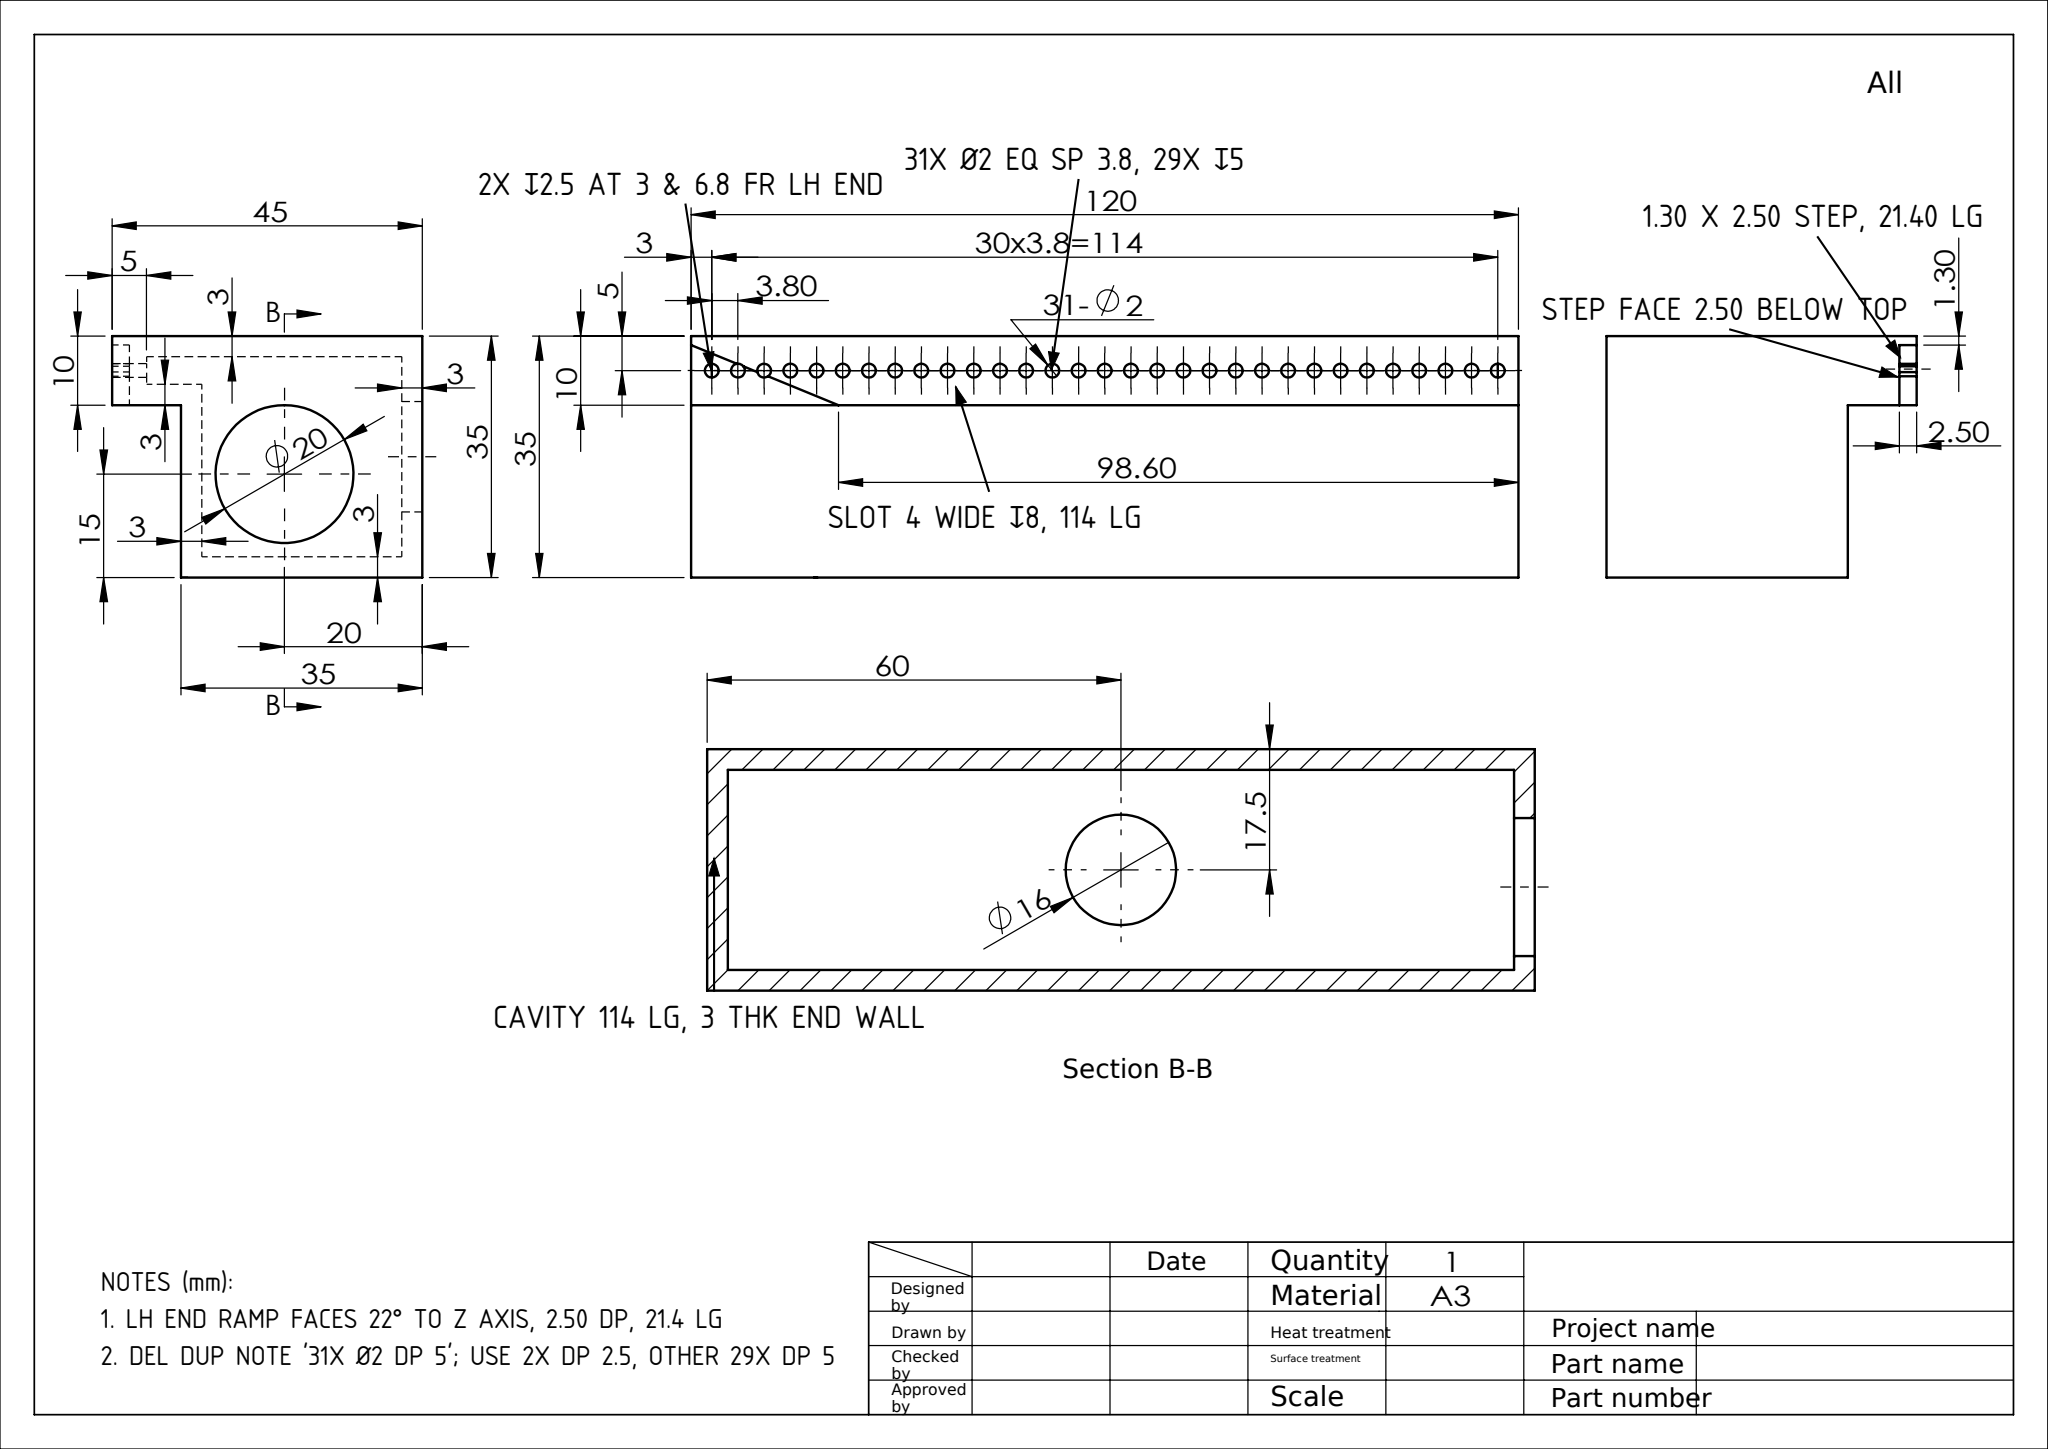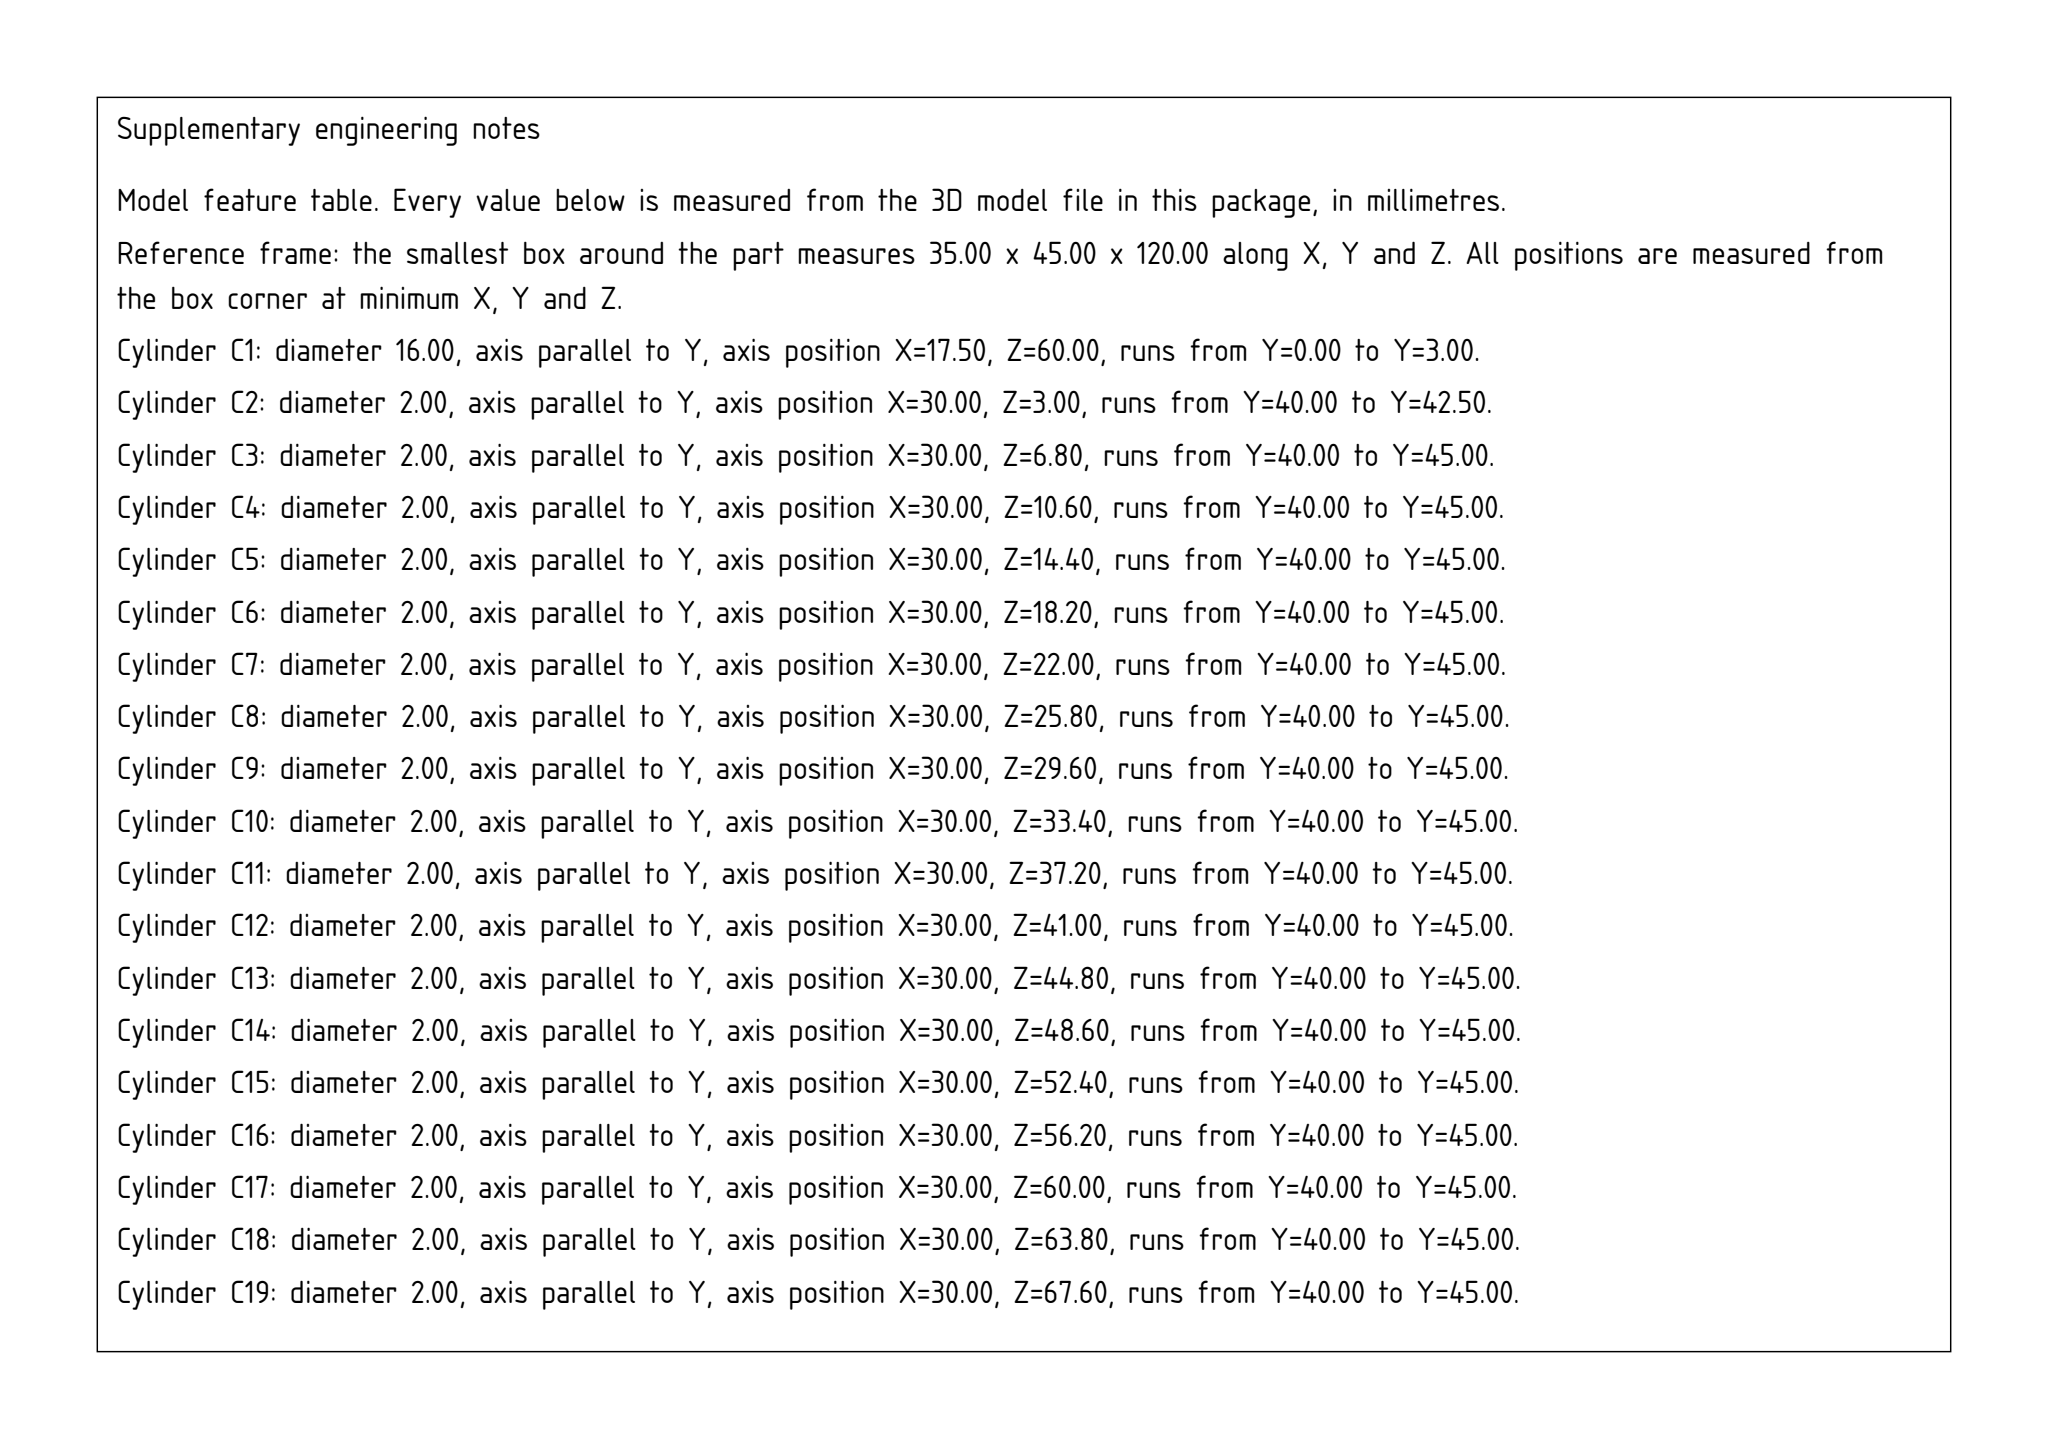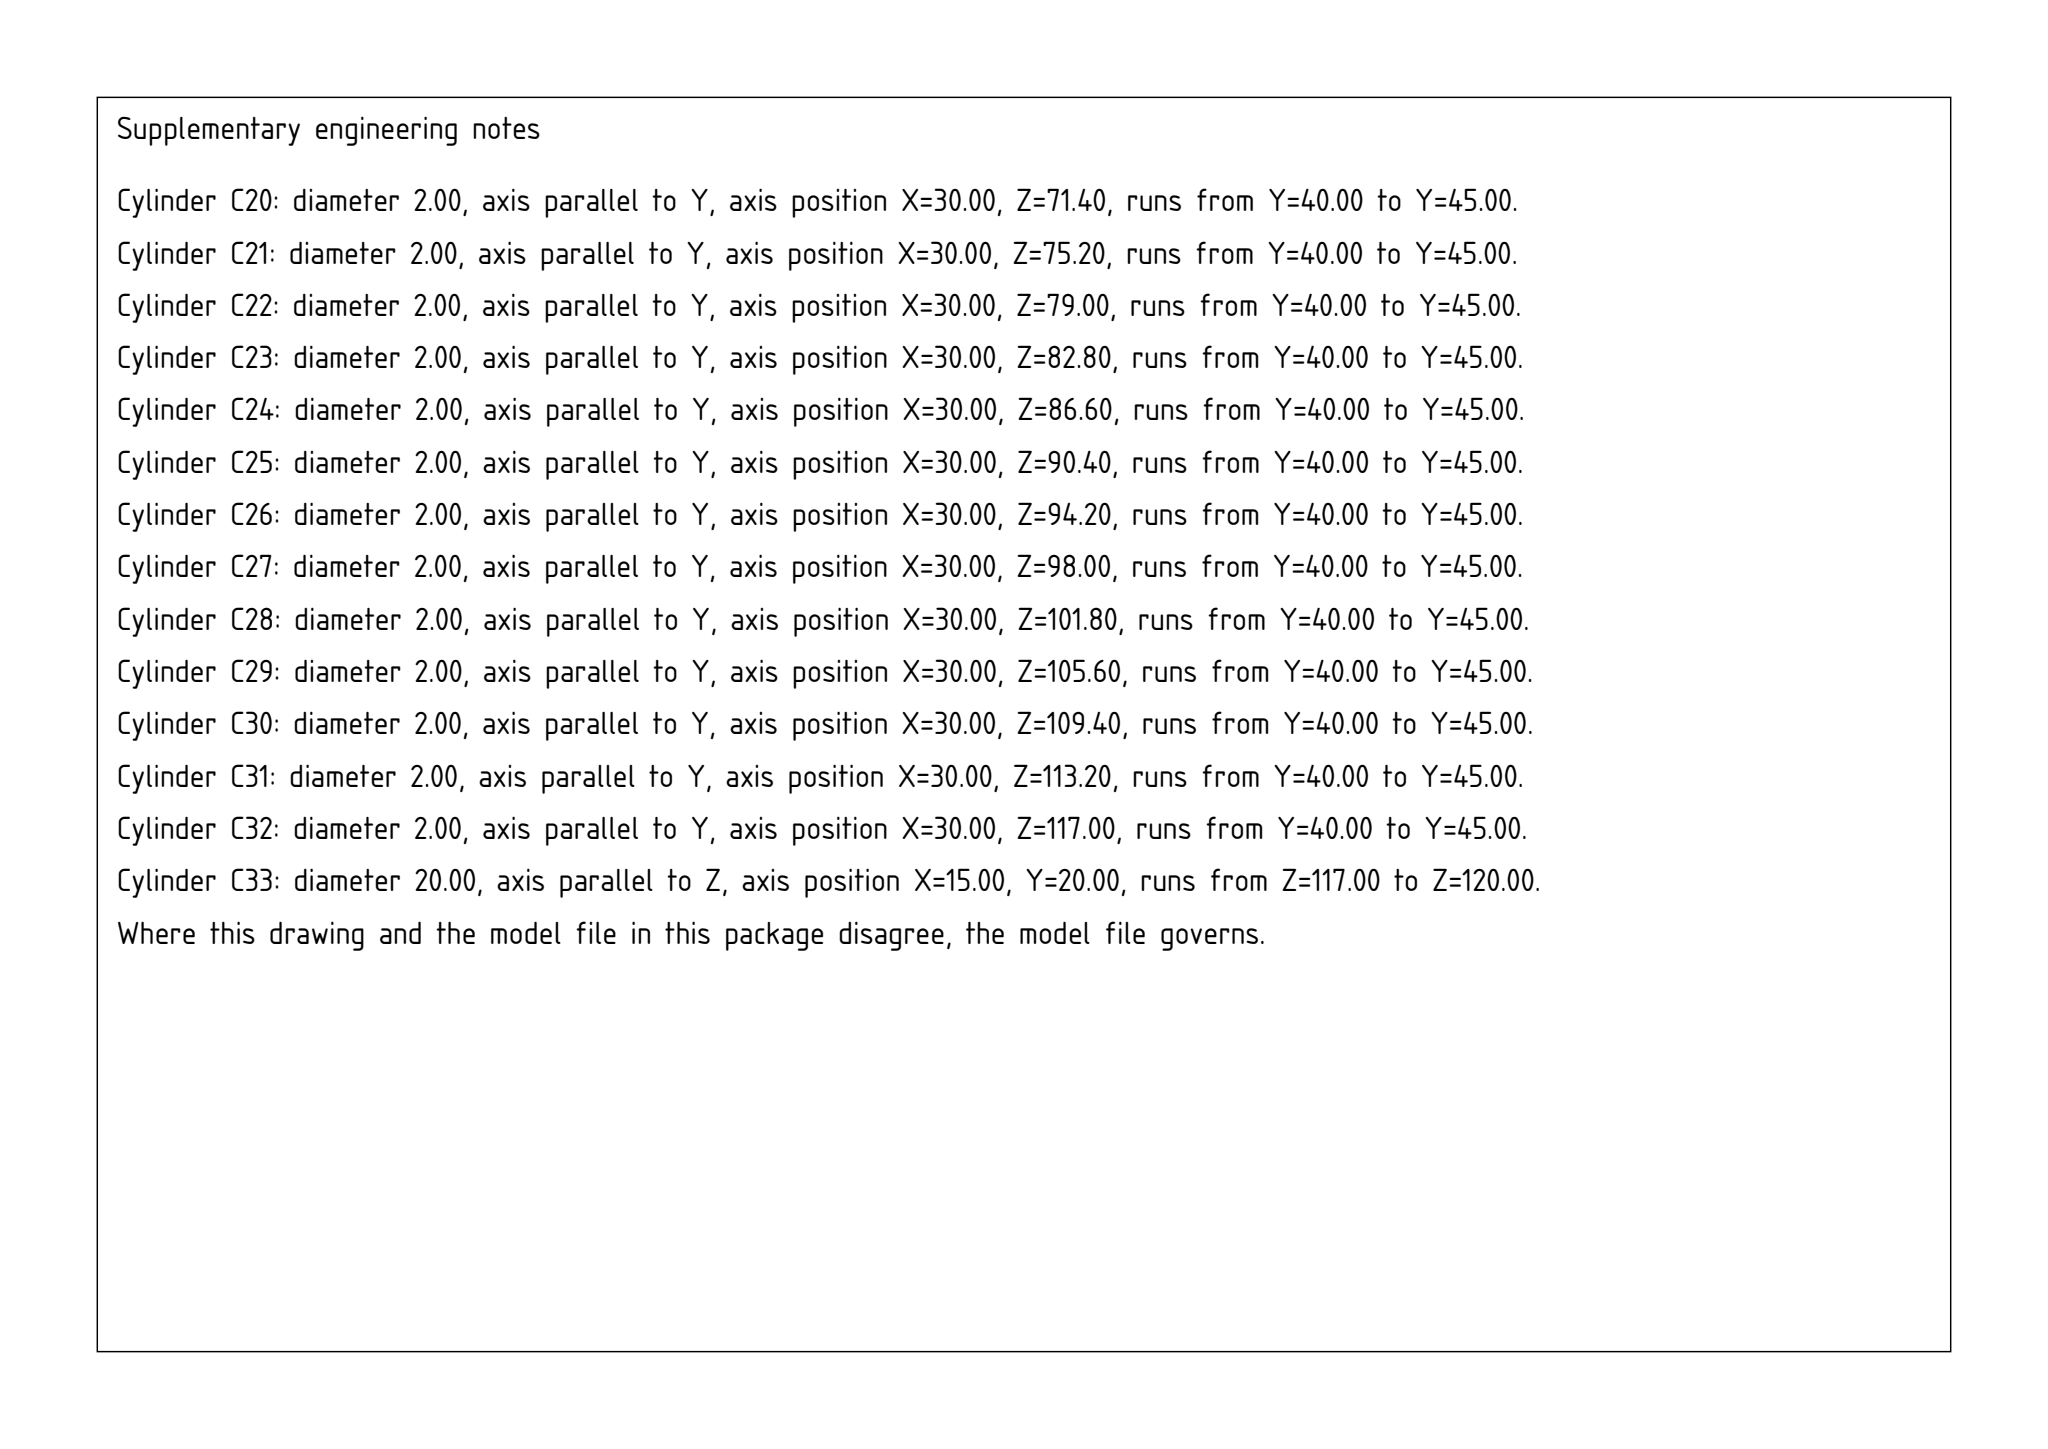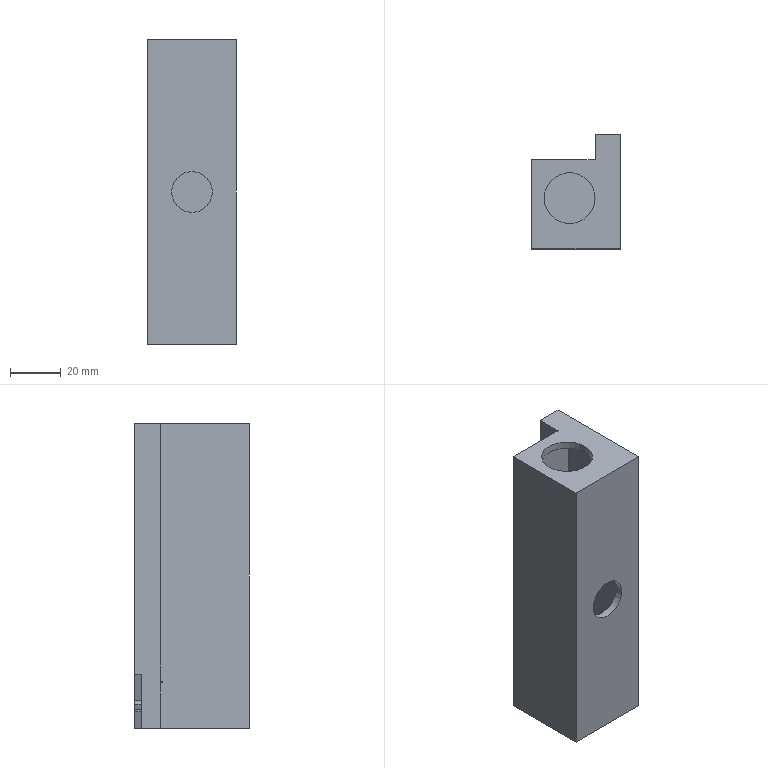Part | SolidWorks | mm | 1 solid | 92 faces | box 35 x 45 x 120 mm | volume 57229 mm3 | cylinder 66 | plane 26 | commonest cylinder face diameters 2 x62 16 x2 20 x2
Drawing notes:
1.30 X 2.50 STEP AT LEFT END FACE: Z=0 TO 21.40 | from the solid: Face y=42.5 (2.50 below y=45 top) spans z 0-21.4, x 25-33.7; 35-33.7=1.30 step seen in left-end view
HOLES AT 3 & 6.8 FR LEFT END ARE DP 2.5; OTHER 29 ARE DP 5 | from the solid: Ø2 cyls at z=3.0 and z=6.8 run y40-42.5 (2.5 deep); all other Ø2 holes run y40-45 (5 deep)
SLOT UNDER Ø2 HOLES: 4 WIDE x 8 DP FROM CAVITY ROOF, 114 LG | from the solid: planes x=28 & x=32 (y 32-40, z 3-117) bound 4 wide channel; roof y=40 vs cavity top y=32 = 8 deep; z 3-117 = 114
INT CAVITY 114 LG, 3 THK END WALL EA END - SECT B-B | from the solid: cavity faces z=3 and z=117 (29x37 section); bbox z 0-120 gives 3 mm end walls, 114 cavity length
LH END RAMP FACES 22° TO Z AXIS, 2.50 DP, 21.4 LG | from the solid: inclined planes angle_to_xyz [22.1,90,67.9] at y 42.5-45 (2.5), x 25-33.7, z 0-21.4
31X Ø2 EQ SP 3.8: 29X DP 5 INTO SLOT, 2X DP 2.5 AT LH RAMP | from the solid: 29 Ø2 bores y 40-45 (5 dp); holes at z=3.0 and z=6.8 run y 40-42.5 (2.5 dp); pitch 3.8, 30x3.8=114
DEL DUP NOTE '31X Ø2 DP 5'; USE 2X DP 2.5, OTHER 29X DP 5 | from the solid: only 2 shallow bores (z=3.0, 6.8) go y 40-42.5; all others y 40-45, so single-depth callout is false
STEP FACE 2.50 BELOW 45 TOP FACE; DEL '0.10 FROM X DATUM' | from the solid: plane y=42.5 (x 25-33.7) vs top face y=45 = 2.50; x=0.1 face is 0 area sliver, no datum
build123d program:
from build123d import *

# Parameters (mm, degrees)
EXTRUDE1_DEPTH     = 120
SKETCH2_R          = 10
CUT_EXTRUDE1_DEPTH = 133.853
CUT_EXTRUDE2_DEPTH = 133.853
SKETCH4_R          = 1
CUT_EXTRUDE3_DEPTH = 5
EXTRUDE2_DEPTH     = 3
EXTRUDE3_DEPTH     = 3
SKETCH8_R          = 10
CUT_EXTRUDE4_DEPTH = 3
CUT_EXTRUDE5_DEPTH = 2.5
CUT_EXTRUDE6_DEPTH = 1
SKETCH11_R         = 8
CUT_EXTRUDE7_DEPTH = 3


with BuildPart() as part:
    # Sketch1 → Extrude1 (new body)
    with BuildSketch(Plane.XY):
        Polygon((0, 0), (0, 35), (25, 35), (25, 45), (35, 45), (35, 0), align=None)
    extrude(amount=EXTRUDE1_DEPTH)

    # Sketch2 → Cut-Extrude1 (cut, through all)
    with BuildSketch(Plane.XY.offset(120)):
        with Locations((20, 20)):
            Circle(SKETCH2_R)
    extrude(amount=-CUT_EXTRUDE1_DEPTH, mode=Mode.SUBTRACT)

    # Sketch3 → Cut-Extrude2 (cut, through all)
    with BuildSketch(Plane.XY.offset(120)):
        Polygon((3, 3), (3, 32), (28, 32), (28, 40), (32, 40), (32, 3), align=None)
    extrude(amount=-CUT_EXTRUDE2_DEPTH, mode=Mode.SUBTRACT)

    # Sketch4 → Cut-Extrude3 (cut)
    with BuildSketch(Plane(origin=(0, 45, 0), x_dir=(1, 0, 0), z_dir=(0, 1, 0))):
        with Locations(Location((30, -3, 0), (0, 0, 270))):
            Circle(SKETCH4_R)
        with Locations(Location((30, -6.8, 0), (0, 0, 270))):
            Circle(SKETCH4_R)
        with Locations(Location((30, -10.6, 0), (0, 0, 270))):
            Circle(SKETCH4_R)
        with Locations(Location((30, -14.4, 0), (0, 0, 270))):
            Circle(SKETCH4_R)
        with Locations(Location((30, -18.2, 0), (0, 0, 270))):
            Circle(SKETCH4_R)
        with Locations(Location((30, -22, 0), (0, 0, 270))):
            Circle(SKETCH4_R)
        with Locations(Location((30, -25.8, 0), (0, 0, 270))):
            Circle(SKETCH4_R)
        with Locations(Location((30, -29.6, 0), (0, 0, 270))):
            Circle(SKETCH4_R)
        with Locations(Location((30, -33.4, 0), (0, 0, 270))):
            Circle(SKETCH4_R)
        with Locations(Location((30, -37.2, 0), (0, 0, 270))):
            Circle(SKETCH4_R)
        with Locations(Location((30, -41, 0), (0, 0, 270))):
            Circle(SKETCH4_R)
        with Locations(Location((30, -44.8, 0), (0, 0, 270))):
            Circle(SKETCH4_R)
        with Locations(Location((30, -48.6, 0), (0, 0, 270))):
            Circle(SKETCH4_R)
        with Locations(Location((30, -52.4, 0), (0, 0, 270))):
            Circle(SKETCH4_R)
        with Locations(Location((30, -56.2, 0), (0, 0, 270))):
            Circle(SKETCH4_R)
        with Locations(Location((30, -60, 0), (0, 0, 270))):
            Circle(SKETCH4_R)
        with Locations(Location((30, -63.8, 0), (0, 0, 270))):
            Circle(SKETCH4_R)
        with Locations(Location((30, -67.6, 0), (0, 0, 270))):
            Circle(SKETCH4_R)
        with Locations(Location((30, -71.4, 0), (0, 0, 270))):
            Circle(SKETCH4_R)
        with Locations(Location((30, -75.2, 0), (0, 0, 270))):
            Circle(SKETCH4_R)
        with Locations(Location((30, -79, 0), (0, 0, 270))):
            Circle(SKETCH4_R)
        with Locations(Location((30, -82.8, 0), (0, 0, 270))):
            Circle(SKETCH4_R)
        with Locations(Location((30, -86.6, 0), (0, 0, 270))):
            Circle(SKETCH4_R)
        with Locations(Location((30, -90.4, 0), (0, 0, 270))):
            Circle(SKETCH4_R)
        with Locations(Location((30, -94.2, 0), (0, 0, 270))):
            Circle(SKETCH4_R)
        with Locations(Location((30, -98, 0), (0, 0, 270))):
            Circle(SKETCH4_R)
        with Locations(Location((30, -101.8, 0), (0, 0, 270))):
            Circle(SKETCH4_R)
        with Locations(Location((30, -105.6, 0), (0, 0, 270))):
            Circle(SKETCH4_R)
        with Locations(Location((30, -109.4, 0), (0, 0, 270))):
            Circle(SKETCH4_R)
        with Locations(Location((30, -113.2, 0), (0, 0, 270))):
            Circle(SKETCH4_R)
        with Locations(Location((30, -117, 0), (0, 0, 270))):
            Circle(SKETCH4_R)
    extrude(amount=-CUT_EXTRUDE3_DEPTH, mode=Mode.SUBTRACT)

    # Sketch5 → Extrude2 (add)
    with BuildSketch(Plane.XY.offset(120)):
        Polygon((28, 32), (3, 32), (3, 3), (32, 3), (32, 40), (28, 40), align=None)
    extrude(amount=-EXTRUDE2_DEPTH)

    # Sketch6 → Extrude3 (add)
    with BuildSketch(Plane(origin=(0, 0, 0), x_dir=(-1, 0, 0), z_dir=(0, 0, -1))):
        Polygon((-28, 40), (-28, 32), (-3, 32), (-3, 3), (-32, 3), (-32, 40), align=None)
    extrude(amount=-EXTRUDE3_DEPTH)

    # Sketch8 → Cut-Extrude4 (cut)
    with BuildSketch(Plane.XY.offset(120)):
        with Locations((15, 20)):
            Circle(SKETCH8_R)
    extrude(amount=-CUT_EXTRUDE4_DEPTH, mode=Mode.SUBTRACT)

    # Sketch9 → Cut-Extrude5 (cut)
    with BuildSketch(Plane(origin=(0, 45, 0), x_dir=(1, 0, 0), z_dir=(0, 1, 0))):
        Polygon((33.7, 0), (25, -21.4), (25, 0), align=None)
    extrude(amount=-CUT_EXTRUDE5_DEPTH, mode=Mode.SUBTRACT)

    # Sketch10 → Cut-Extrude6 (cut)
    with BuildSketch(Plane(origin=(0, 35, 0), x_dir=(1, 0, 0), z_dir=(0, 1, 0))):
        Polygon((0.05561, -18.3), (0, -18.277), (0, -17.946), (0.05561, -17.946), align=None)
    extrude(amount=-CUT_EXTRUDE6_DEPTH, mode=Mode.SUBTRACT)

    # Sketch11 → Cut-Extrude7 (cut)
    with BuildSketch(Plane.XZ):
        with Locations((17.5, 60)):
            Circle(SKETCH11_R)
    extrude(amount=-CUT_EXTRUDE7_DEPTH, mode=Mode.SUBTRACT)


solid = part.part